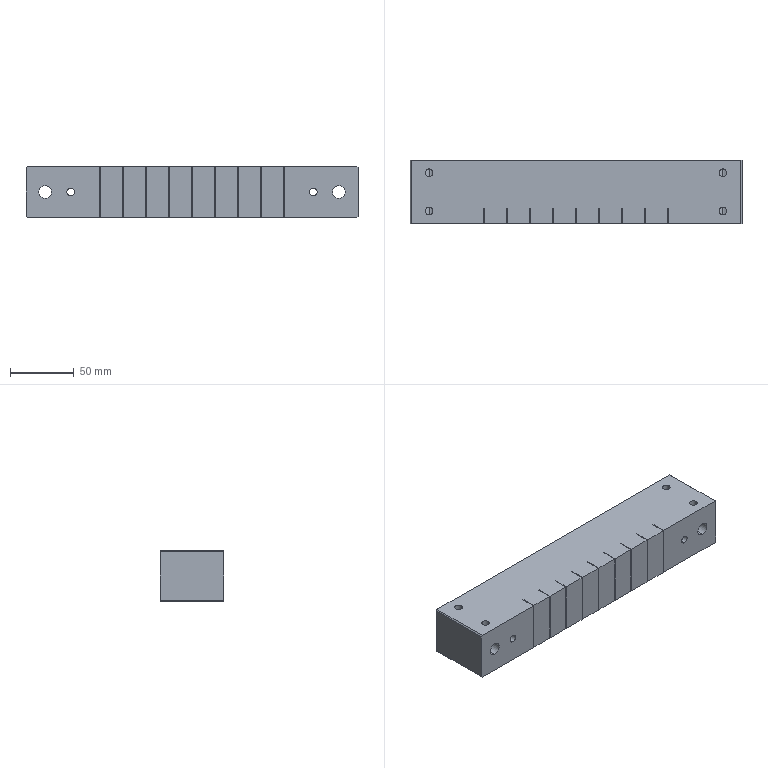Component | SolidWorks | 8TC-A15004-60-26A-1 | 1 solid | 62 faces | box 260 x 50 x 40 mm | volume 505335 mm3 | plane 46 | cylinder 16 | commonest cylinder face diameters 6 x12 10 x4 | material Cr12
build123d program:
from build123d import *

# Parameters (mm, degrees)
SKETCH1_W              = 260
SKETCH1_H              = 40
BOSS_EXTRUDE1_DEPTH    = 25
SKETCH3_R              = 3
CUT_EXTRUDE2_DEPTH     = 141.712
SKETCH2_W              = 0.5
SKETCH2_H              = 40
CUT_EXTRUDE1_DEPTH     = 12
LPATTERN1_COUNT        = 9
LPATTERN1_PITCH        = 18
SKETCH4_R              = 5
CUT_EXTRUDE3_DEPTH     = 141.712
CHAMFER1_SIZE          = 1
M6_TAPPED_HOLE1_REACH  = 140.293
M6_TAPPED_HOLE1_BORE_R = 3


with BuildPart() as part:
    # Sketch1 → Boss-Extrude1 (new, symmetric)
    with BuildSketch(Plane(origin=(0, 0, 0), x_dir=(1, 0, 0), z_dir=(0, 1, 0))):
        Rectangle(SKETCH1_W, SKETCH1_H)
    extrude(amount=BOSS_EXTRUDE1_DEPTH, both=True)

    # Sketch3 → Cut-Extrude2 (cut, through all)
    with BuildSketch(Plane.XZ.offset(25)):
        with Locations(Location((-95, 0, 0), (0, 0, 270))):
            Circle(SKETCH3_R)
        with Locations(Location((95, 0, 0), (0, 0, 90))):
            Circle(SKETCH3_R)
    extrude(amount=-CUT_EXTRUDE2_DEPTH, mode=Mode.SUBTRACT)

    # Sketch2 → Cut-Extrude1 (cut)
    with BuildSketch(Plane.XZ.offset(25)):
        with Locations((-72, 0)):
            Rectangle(SKETCH2_W, SKETCH2_H)
    cut_extrude1 = extrude(amount=-CUT_EXTRUDE1_DEPTH, mode=Mode.SUBTRACT)

    # LPattern1: Cut-Extrude1 ×9
    with Locations(*[(i * LPATTERN1_PITCH, 0, 0) for i in range(1, LPATTERN1_COUNT)]):
        add(cut_extrude1, mode=Mode.SUBTRACT)

    # Sketch4 → Cut-Extrude3 (cut, through all)
    with BuildSketch(Plane.XZ.offset(25)):
        with Locations(Location((-115, 0, 0), (0, 0, 270))):
            Circle(SKETCH4_R)
        with Locations(Location((115, 0, 0), (0, 0, 90))):
            Circle(SKETCH4_R)
    extrude(amount=-CUT_EXTRUDE3_DEPTH, mode=Mode.SUBTRACT)

    # Chamfer1
    chamfer1_edges = [part.edges().sort_by_distance(p)[0] for p in [
        (130, 0, 20),
        (-130, 0, 20),
        (-130, 0, -20),
        (130, 0, -20),
    ]]
    chamfer(chamfer1_edges, length=CHAMFER1_SIZE)

    # M6 Tapped Hole1 bore → M6 Tapped Hole1 (cut, up to next)
    with BuildSketch(Plane(origin=(0, 0, -20), x_dir=(-1, 0, 0), z_dir=(0, 0, -1)), mode=Mode.PRIVATE) as m6_tapped_hole1_sk1:
        with Locations((-115, 15)):
            Circle(M6_TAPPED_HOLE1_BORE_R)
    m6_tapped_hole1_tool1 = extrude(m6_tapped_hole1_sk1.sketch, amount=-M6_TAPPED_HOLE1_REACH, mode=Mode.PRIVATE) & part.part
    # M6 Tapped Hole1 bore → M6 Tapped Hole1 (cut, up to next)
    with BuildSketch(Plane(origin=(0, 0, -20), x_dir=(-1, 0, 0), z_dir=(0, 0, -1)), mode=Mode.PRIVATE) as m6_tapped_hole1_sk2:
        with Locations((-115, -15)):
            Circle(M6_TAPPED_HOLE1_BORE_R)
    m6_tapped_hole1_tool2 = extrude(m6_tapped_hole1_sk2.sketch, amount=-M6_TAPPED_HOLE1_REACH, mode=Mode.PRIVATE) & part.part
    # M6 Tapped Hole1 bore → M6 Tapped Hole1 (cut, up to next)
    with BuildSketch(Plane(origin=(0, 0, -20), x_dir=(-1, 0, 0), z_dir=(0, 0, -1)), mode=Mode.PRIVATE) as m6_tapped_hole1_sk3:
        with Locations((115, -15)):
            Circle(M6_TAPPED_HOLE1_BORE_R)
    m6_tapped_hole1_tool3 = extrude(m6_tapped_hole1_sk3.sketch, amount=-M6_TAPPED_HOLE1_REACH, mode=Mode.PRIVATE) & part.part
    # M6 Tapped Hole1 bore → M6 Tapped Hole1 (cut, up to next)
    with BuildSketch(Plane(origin=(0, 0, -20), x_dir=(-1, 0, 0), z_dir=(0, 0, -1)), mode=Mode.PRIVATE) as m6_tapped_hole1_sk4:
        with Locations((115, 15)):
            Circle(M6_TAPPED_HOLE1_BORE_R)
    m6_tapped_hole1_tool4 = extrude(m6_tapped_hole1_sk4.sketch, amount=-M6_TAPPED_HOLE1_REACH, mode=Mode.PRIVATE) & part.part
    add(m6_tapped_hole1_tool1.solids().sort_by_distance((115, 15, -20))[0], mode=Mode.SUBTRACT)
    add(m6_tapped_hole1_tool2.solids().sort_by_distance((115, -15, -20))[0], mode=Mode.SUBTRACT)
    add(m6_tapped_hole1_tool3.solids().sort_by_distance((-115, -15, -20))[0], mode=Mode.SUBTRACT)
    add(m6_tapped_hole1_tool4.solids().sort_by_distance((-115, 15, -20))[0], mode=Mode.SUBTRACT)


solid = part.part

# Placed as in the assembly
solid = solid.moved(Location((26.714, 0, 0), (-180, 0, 180)))